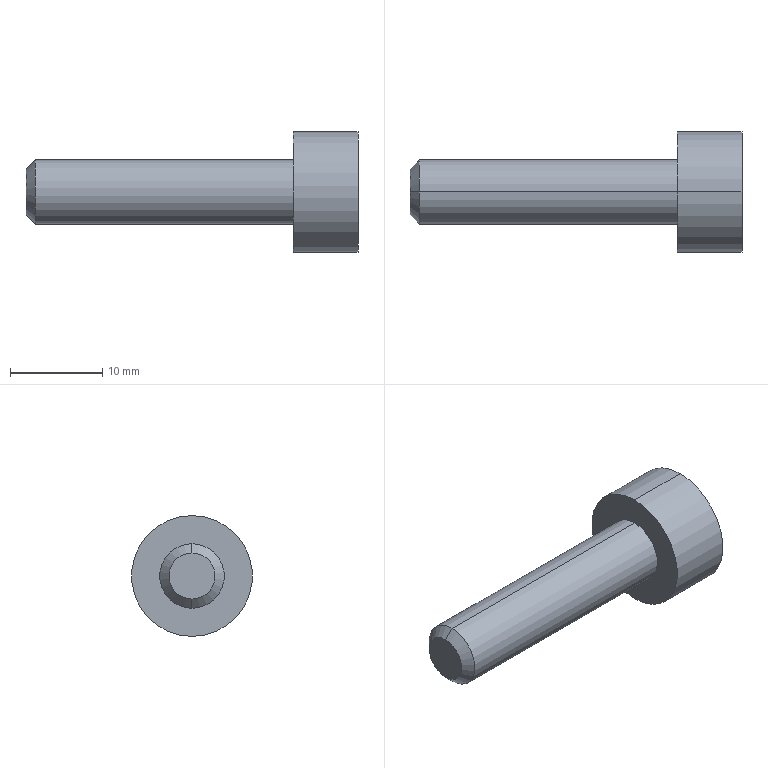Component | SolidWorks | HexSocketScrewM6X15-1 | 1 solid | 16 faces | box 36 x 13.09 x 13.09 mm | volume 1927 mm3 | plane 10 | cylinder 4 | cone 2 | commonest cylinder face diameters 13.093 x2 7 x2
build123d program:
from build123d import *

# Parameters (mm, degrees)
SKETCH2_R           = 3.5
BOSS_EXTRUDE1_DEPTH = 29
SKETCH3_R           = 6.547
BOSS_EXTRUDE2_DEPTH = 7
CHAMFER1_SIZE       = 1
CUT_EXTRUDE1_DEPTH  = 3


with BuildPart() as part:
    # Sketch2 → Boss-Extrude1 (new body)
    with BuildSketch(Plane.XY):
        with Locations((0, 12.224)):
            Circle(SKETCH2_R)
    extrude(amount=-BOSS_EXTRUDE1_DEPTH)

    # Sketch3 → Boss-Extrude2 (add)
    with BuildSketch(Plane.XY):
        with Locations((0, 12.224)):
            Circle(SKETCH3_R)
    extrude(amount=BOSS_EXTRUDE2_DEPTH)

    # Chamfer1
    chamfer1_edges = [part.edges().sort_by_distance(p)[0] for p in [
        (-3.5, 12.224, -29),
    ]]
    chamfer(chamfer1_edges, length=CHAMFER1_SIZE)

    # Sketch4 → Cut-Extrude1 (cut)
    with BuildSketch(Plane.XY.offset(7)):
        Polygon((0.1708, 16.162), (-3.326, 14.341), (-3.496, 10.402), (-0.1708, 8.285), (3.326, 10.106), (3.496, 14.045), align=None)
    extrude(amount=-CUT_EXTRUDE1_DEPTH, mode=Mode.SUBTRACT)


solid = part.part

# Placed as in the assembly
solid = solid.moved(Location((-277, 0, 0), (0, 90, 0)))
STEP:
#1=COLOUR_RGB('',0.7922,0.8196,0.9333);
#2=FILL_AREA_STYLE_COLOUR('',#1);
#3=FILL_AREA_STYLE('',(#2));
#4=SURFACE_STYLE_FILL_AREA(#3);
#5=SURFACE_SIDE_STYLE('',(#4));
#6=SURFACE_STYLE_USAGE(.BOTH.,#5);
#7=PRESENTATION_STYLE_ASSIGNMENT((#6));
#8=CARTESIAN_POINT('',(-12.047,0.4812,0.09843));
#9=VERTEX_POINT('',#8);
#10=CARTESIAN_POINT('',(-12.047,0.4812,-0.09843));
#11=VERTEX_POINT('',#10);
#12=CARTESIAN_POINT('',(-12.047,0.4812,-0.));
#13=DIRECTION('',(-1.,0.,0.));
#14=DIRECTION('',(0.,0.,-1.));
#15=AXIS2_PLACEMENT_3D('',#12,#13,#14);
#16=CIRCLE('',#15,0.09843);
#17=EDGE_CURVE('',#9,#11,#16,.T.);
#18=ORIENTED_EDGE('',*,*,#17,.F.);
#19=CARTESIAN_POINT('',(-12.008,0.4812,0.1378));
#20=VERTEX_POINT('',#19);
#21=CARTESIAN_POINT('',(-12.008,0.4812,0.1378));
#22=DIRECTION('',(0.7071,0.,0.7071));
#23=VECTOR('',#22,39.37);
#24=LINE('',#21,#23);
#25=EDGE_CURVE('',#9,#20,#24,.T.);
#26=ORIENTED_EDGE('',*,*,#25,.T.);
#27=CARTESIAN_POINT('',(-12.008,0.4812,-0.1378));
#28=VERTEX_POINT('',#27);
#29=CARTESIAN_POINT('',(-12.008,0.4812,-0.));
#30=DIRECTION('',(1.,0.,0.));
#31=DIRECTION('',(0.,0.,-1.));
#32=AXIS2_PLACEMENT_3D('',#29,#30,#31);
#33=CIRCLE('',#32,0.1378);
#34=EDGE_CURVE('',#28,#20,#33,.T.);
#35=ORIENTED_EDGE('',*,*,#34,.F.);
#36=CARTESIAN_POINT('',(-12.008,0.4812,-0.1378));
#37=DIRECTION('',(0.7071,0.,-0.7071));
#38=VECTOR('',#37,39.37);
#39=LINE('',#36,#38);
#40=EDGE_CURVE('',#11,#28,#39,.T.);
#41=ORIENTED_EDGE('',*,*,#40,.F.);
#42=EDGE_LOOP('',(#18,#26,#35,#41));
#43=FACE_OUTER_BOUND('',#42,.T.);
#44=CARTESIAN_POINT('',(-12.008,0.4812,-0.));
#45=DIRECTION('',(1.,0.,0.));
#46=DIRECTION('',(0.,0.,-1.));
#47=AXIS2_PLACEMENT_3D('',#44,#45,#46);
#48=CONICAL_SURFACE('',#47,0.1378,0.7854);
#49=ADVANCED_FACE('',(#43),#48,.T.);
#50=CARTESIAN_POINT('',(-10.63,0.4812,-0.2577));
#51=VERTEX_POINT('',#50);
#52=CARTESIAN_POINT('',(-10.63,0.4812,0.2577));
#53=VERTEX_POINT('',#52);
#54=CARTESIAN_POINT('',(-10.63,0.4812,0.));
#55=DIRECTION('',(1.,0.,0.));
#56=DIRECTION('',(0.,0.,-1.));
#57=AXIS2_PLACEMENT_3D('',#54,#55,#56);
#58=CIRCLE('',#57,0.2577);
#59=EDGE_CURVE('',#51,#53,#58,.T.);
#60=ORIENTED_EDGE('',*,*,#59,.F.);
#61=CARTESIAN_POINT('',(-10.906,0.4812,-0.2577));
#62=VERTEX_POINT('',#61);
#63=CARTESIAN_POINT('',(-10.63,0.4812,-0.2577));
#64=DIRECTION('',(-1.,0.,0.));
#65=VECTOR('',#64,39.37);
#66=LINE('',#63,#65);
#67=EDGE_CURVE('',#51,#62,#66,.T.);
#68=ORIENTED_EDGE('',*,*,#67,.T.);
#69=CARTESIAN_POINT('',(-10.906,0.4812,0.2577));
#70=VERTEX_POINT('',#69);
#71=CARTESIAN_POINT('',(-10.906,0.4812,0.));
#72=DIRECTION('',(1.,0.,0.));
#73=DIRECTION('',(0.,0.,-1.));
#74=AXIS2_PLACEMENT_3D('',#71,#72,#73);
#75=CIRCLE('',#74,0.2577);
#76=EDGE_CURVE('',#62,#70,#75,.T.);
#77=ORIENTED_EDGE('',*,*,#76,.T.);
#78=CARTESIAN_POINT('',(-10.63,0.4812,0.2577));
#79=DIRECTION('',(-1.,0.,0.));
#80=VECTOR('',#79,39.37);
#81=LINE('',#78,#80);
#82=EDGE_CURVE('',#53,#70,#81,.T.);
#83=ORIENTED_EDGE('',*,*,#82,.F.);
#84=EDGE_LOOP('',(#60,#68,#77,#83));
#85=FACE_OUTER_BOUND('',#84,.T.);
#86=CARTESIAN_POINT('',(-10.63,0.4812,0.));
#87=DIRECTION('',(-1.,0.,0.));
#88=DIRECTION('',(0.,0.,1.));
#89=AXIS2_PLACEMENT_3D('',#86,#87,#88);
#90=CYLINDRICAL_SURFACE('',#89,0.2577);
#91=ADVANCED_FACE('',(#85),#90,.T.);
#92=ORIENTED_EDGE('',*,*,#34,.T.);
#93=CARTESIAN_POINT('',(-10.906,0.4812,0.1378));
#94=VERTEX_POINT('',#93);
#95=CARTESIAN_POINT('',(-12.047,0.4812,0.1378));
#96=DIRECTION('',(1.,0.,0.));
#97=VECTOR('',#96,39.37);
#98=LINE('',#95,#97);
#99=EDGE_CURVE('',#20,#94,#98,.T.);
#100=ORIENTED_EDGE('',*,*,#99,.T.);
#101=CARTESIAN_POINT('',(-10.906,0.4812,-0.1378));
#102=VERTEX_POINT('',#101);
#103=CARTESIAN_POINT('',(-10.906,0.4812,-0.));
#104=DIRECTION('',(1.,0.,0.));
#105=DIRECTION('',(0.,0.,-1.));
#106=AXIS2_PLACEMENT_3D('',#103,#104,#105);
#107=CIRCLE('',#106,0.1378);
#108=EDGE_CURVE('',#102,#94,#107,.T.);
#109=ORIENTED_EDGE('',*,*,#108,.F.);
#110=CARTESIAN_POINT('',(-12.047,0.4812,-0.1378));
#111=DIRECTION('',(1.,0.,0.));
#112=VECTOR('',#111,39.37);
#113=LINE('',#110,#112);
#114=EDGE_CURVE('',#28,#102,#113,.T.);
#115=ORIENTED_EDGE('',*,*,#114,.F.);
#116=EDGE_LOOP('',(#92,#100,#109,#115));
#117=FACE_OUTER_BOUND('',#116,.T.);
#118=CARTESIAN_POINT('',(-12.047,0.4812,-0.));
#119=DIRECTION('',(1.,0.,0.));
#120=DIRECTION('',(0.,0.,-1.));
#121=AXIS2_PLACEMENT_3D('',#118,#119,#120);
#122=CYLINDRICAL_SURFACE('',#121,0.1378);
#123=ADVANCED_FACE('',(#117),#122,.T.);
#124=ORIENTED_EDGE('',*,*,#99,.F.);
#125=CARTESIAN_POINT('',(-12.008,0.4812,-0.));
#126=DIRECTION('',(1.,0.,0.));
#127=DIRECTION('',(0.,0.,-1.));
#128=AXIS2_PLACEMENT_3D('',#125,#126,#127);
#129=CIRCLE('',#128,0.1378);
#130=EDGE_CURVE('',#20,#28,#129,.T.);
#131=ORIENTED_EDGE('',*,*,#130,.T.);
#132=ORIENTED_EDGE('',*,*,#114,.T.);
#133=CARTESIAN_POINT('',(-10.906,0.4812,-0.));
#134=DIRECTION('',(1.,0.,0.));
#135=DIRECTION('',(0.,0.,-1.));
#136=AXIS2_PLACEMENT_3D('',#133,#134,#135);
#137=CIRCLE('',#136,0.1378);
#138=EDGE_CURVE('',#94,#102,#137,.T.);
#139=ORIENTED_EDGE('',*,*,#138,.F.);
#140=EDGE_LOOP('',(#124,#131,#132,#139));
#141=FACE_OUTER_BOUND('',#140,.T.);
#142=CARTESIAN_POINT('',(-12.047,0.4812,-0.));
#143=DIRECTION('',(1.,0.,0.));
#144=DIRECTION('',(0.,0.,-1.));
#145=AXIS2_PLACEMENT_3D('',#142,#143,#144);
#146=CYLINDRICAL_SURFACE('',#145,0.1378);
#147=ADVANCED_FACE('',(#141),#146,.T.);
#148=CARTESIAN_POINT('',(-12.047,0.4812,-0.));
#149=DIRECTION('',(-1.,0.,0.));
#150=DIRECTION('',(0.,0.,-1.));
#151=AXIS2_PLACEMENT_3D('',#148,#149,#150);
#152=CIRCLE('',#151,0.09843);
#153=EDGE_CURVE('',#11,#9,#152,.T.);
#154=ORIENTED_EDGE('',*,*,#153,.T.);
#155=ORIENTED_EDGE('',*,*,#17,.T.);
#156=EDGE_LOOP('',(#154,#155));
#157=FACE_OUTER_BOUND('',#156,.T.);
#158=CARTESIAN_POINT('',(-12.047,0.4812,-0.));
#159=DIRECTION('',(1.,0.,0.));
#160=DIRECTION('',(0.,0.,-1.));
#161=AXIS2_PLACEMENT_3D('',#158,#159,#160);
#162=PLANE('',#161);
#163=ADVANCED_FACE('',(#157),#162,.F.);
#164=ORIENTED_EDGE('',*,*,#67,.F.);
#165=CARTESIAN_POINT('',(-10.63,0.4812,0.));
#166=DIRECTION('',(1.,0.,0.));
#167=DIRECTION('',(0.,0.,-1.));
#168=AXIS2_PLACEMENT_3D('',#165,#166,#167);
#169=CIRCLE('',#168,0.2577);
#170=EDGE_CURVE('',#53,#51,#169,.T.);
#171=ORIENTED_EDGE('',*,*,#170,.F.);
#172=ORIENTED_EDGE('',*,*,#82,.T.);
#173=CARTESIAN_POINT('',(-10.906,0.4812,0.));
#174=DIRECTION('',(1.,0.,0.));
#175=DIRECTION('',(0.,0.,-1.));
#176=AXIS2_PLACEMENT_3D('',#173,#174,#175);
#177=CIRCLE('',#176,0.2577);
#178=EDGE_CURVE('',#70,#62,#177,.T.);
#179=ORIENTED_EDGE('',*,*,#178,.T.);
#180=EDGE_LOOP('',(#164,#171,#172,#179));
#181=FACE_OUTER_BOUND('',#180,.T.);
#182=CARTESIAN_POINT('',(-10.63,0.4812,0.));
#183=DIRECTION('',(-1.,0.,0.));
#184=DIRECTION('',(0.,0.,1.));
#185=AXIS2_PLACEMENT_3D('',#182,#183,#184);
#186=CYLINDRICAL_SURFACE('',#185,0.2577);
#187=ADVANCED_FACE('',(#181),#186,.T.);
#188=CARTESIAN_POINT('',(-10.63,0.553,-0.1377));
#189=VERTEX_POINT('',#188);
#190=CARTESIAN_POINT('',(-10.63,0.6363,-0.006726));
#191=VERTEX_POINT('',#190);
#192=CARTESIAN_POINT('',(-10.63,0.553,-0.1377));
#193=DIRECTION('',(0.,0.5371,0.8435));
#194=VECTOR('',#193,39.37);
#195=LINE('',#192,#194);
#196=EDGE_CURVE('',#189,#191,#195,.T.);
#197=ORIENTED_EDGE('',*,*,#196,.F.);
#198=CARTESIAN_POINT('',(-10.63,0.3979,-0.1309));
#199=VERTEX_POINT('',#198);
#200=CARTESIAN_POINT('',(-10.63,0.3979,-0.1309));
#201=DIRECTION('',(0.,0.9991,-0.04333));
#202=VECTOR('',#201,39.37);
#203=LINE('',#200,#202);
#204=EDGE_CURVE('',#199,#189,#203,.T.);
#205=ORIENTED_EDGE('',*,*,#204,.F.);
#206=CARTESIAN_POINT('',(-10.63,0.3262,0.006726));
#207=VERTEX_POINT('',#206);
#208=CARTESIAN_POINT('',(-10.63,0.3262,0.006726));
#209=DIRECTION('',(0.,0.462,-0.8869));
#210=VECTOR('',#209,39.37);
#211=LINE('',#208,#210);
#212=EDGE_CURVE('',#207,#199,#211,.T.);
#213=ORIENTED_EDGE('',*,*,#212,.F.);
#214=CARTESIAN_POINT('',(-10.63,0.4095,0.1377));
#215=VERTEX_POINT('',#214);
#216=CARTESIAN_POINT('',(-10.63,0.4095,0.1377));
#217=DIRECTION('',(0.,-0.5371,-0.8435));
#218=VECTOR('',#217,39.37);
#219=LINE('',#216,#218);
#220=EDGE_CURVE('',#215,#207,#219,.T.);
#221=ORIENTED_EDGE('',*,*,#220,.F.);
#222=CARTESIAN_POINT('',(-10.63,0.5646,0.1309));
#223=VERTEX_POINT('',#222);
#224=CARTESIAN_POINT('',(-10.63,0.5646,0.1309));
#225=DIRECTION('',(0.,-0.9991,0.04333));
#226=VECTOR('',#225,39.37);
#227=LINE('',#224,#226);
#228=EDGE_CURVE('',#223,#215,#227,.T.);
#229=ORIENTED_EDGE('',*,*,#228,.F.);
#230=CARTESIAN_POINT('',(-10.63,0.6363,-0.006726));
#231=DIRECTION('',(0.,-0.462,0.8869));
#232=VECTOR('',#231,39.37);
#233=LINE('',#230,#232);
#234=EDGE_CURVE('',#191,#223,#233,.T.);
#235=ORIENTED_EDGE('',*,*,#234,.F.);
#236=EDGE_LOOP('',(#197,#205,#213,#221,#229,#235));
#237=FACE_BOUND('',#236,.T.);
#238=ORIENTED_EDGE('',*,*,#170,.T.);
#239=ORIENTED_EDGE('',*,*,#59,.T.);
#240=EDGE_LOOP('',(#238,#239));
#241=FACE_OUTER_BOUND('',#240,.T.);
#242=CARTESIAN_POINT('',(-10.63,0.4812,0.));
#243=DIRECTION('',(1.,0.,0.));
#244=DIRECTION('',(0.,0.,-1.));
#245=AXIS2_PLACEMENT_3D('',#242,#243,#244);
#246=PLANE('',#245);
#247=ADVANCED_FACE('',(#237,#241),#246,.T.);
#248=ORIENTED_EDGE('',*,*,#108,.T.);
#249=ORIENTED_EDGE('',*,*,#138,.T.);
#250=EDGE_LOOP('',(#248,#249));
#251=FACE_BOUND('',#250,.T.);
#252=ORIENTED_EDGE('',*,*,#178,.F.);
#253=ORIENTED_EDGE('',*,*,#76,.F.);
#254=EDGE_LOOP('',(#252,#253));
#255=FACE_OUTER_BOUND('',#254,.T.);
#256=CARTESIAN_POINT('',(-10.906,0.4812,0.));
#257=DIRECTION('',(1.,0.,0.));
#258=DIRECTION('',(0.,0.,-1.));
#259=AXIS2_PLACEMENT_3D('',#256,#257,#258);
#260=PLANE('',#259);
#261=ADVANCED_FACE('',(#251,#255),#260,.F.);
#262=ORIENTED_EDGE('',*,*,#25,.F.);
#263=ORIENTED_EDGE('',*,*,#153,.F.);
#264=ORIENTED_EDGE('',*,*,#40,.T.);
#265=ORIENTED_EDGE('',*,*,#130,.F.);
#266=EDGE_LOOP('',(#262,#263,#264,#265));
#267=FACE_OUTER_BOUND('',#266,.T.);
#268=CARTESIAN_POINT('',(-12.008,0.4812,-0.));
#269=DIRECTION('',(1.,0.,0.));
#270=DIRECTION('',(0.,0.,-1.));
#271=AXIS2_PLACEMENT_3D('',#268,#269,#270);
#272=CONICAL_SURFACE('',#271,0.1378,0.7854);
#273=ADVANCED_FACE('',(#267),#272,.T.);
#274=ORIENTED_EDGE('',*,*,#196,.T.);
#275=CARTESIAN_POINT('',(-10.748,0.6363,-0.006726));
#276=VERTEX_POINT('',#275);
#277=CARTESIAN_POINT('',(-10.748,0.6363,-0.006726));
#278=DIRECTION('',(1.,0.,0.));
#279=VECTOR('',#278,39.37);
#280=LINE('',#277,#279);
#281=EDGE_CURVE('',#276,#191,#280,.T.);
#282=ORIENTED_EDGE('',*,*,#281,.F.);
#283=CARTESIAN_POINT('',(-10.748,0.553,-0.1377));
#284=VERTEX_POINT('',#283);
#285=CARTESIAN_POINT('',(-10.748,0.553,-0.1377));
#286=DIRECTION('',(0.,0.5371,0.8435));
#287=VECTOR('',#286,39.37);
#288=LINE('',#285,#287);
#289=EDGE_CURVE('',#284,#276,#288,.T.);
#290=ORIENTED_EDGE('',*,*,#289,.F.);
#291=CARTESIAN_POINT('',(-10.748,0.553,-0.1377));
#292=DIRECTION('',(1.,0.,0.));
#293=VECTOR('',#292,39.37);
#294=LINE('',#291,#293);
#295=EDGE_CURVE('',#284,#189,#294,.T.);
#296=ORIENTED_EDGE('',*,*,#295,.T.);
#297=EDGE_LOOP('',(#274,#282,#290,#296));
#298=FACE_OUTER_BOUND('',#297,.T.);
#299=CARTESIAN_POINT('',(-10.748,0.553,-0.1377));
#300=DIRECTION('',(0.,0.8435,-0.5371));
#301=DIRECTION('',(0.,0.5371,0.8435));
#302=AXIS2_PLACEMENT_3D('',#299,#300,#301);
#303=PLANE('',#302);
#304=ADVANCED_FACE('',(#298),#303,.F.);
#305=ORIENTED_EDGE('',*,*,#204,.T.);
#306=ORIENTED_EDGE('',*,*,#295,.F.);
#307=CARTESIAN_POINT('',(-10.748,0.3979,-0.1309));
#308=VERTEX_POINT('',#307);
#309=CARTESIAN_POINT('',(-10.748,0.3979,-0.1309));
#310=DIRECTION('',(0.,0.9991,-0.04333));
#311=VECTOR('',#310,39.37);
#312=LINE('',#309,#311);
#313=EDGE_CURVE('',#308,#284,#312,.T.);
#314=ORIENTED_EDGE('',*,*,#313,.F.);
#315=CARTESIAN_POINT('',(-10.748,0.3979,-0.1309));
#316=DIRECTION('',(1.,0.,0.));
#317=VECTOR('',#316,39.37);
#318=LINE('',#315,#317);
#319=EDGE_CURVE('',#308,#199,#318,.T.);
#320=ORIENTED_EDGE('',*,*,#319,.T.);
#321=EDGE_LOOP('',(#305,#306,#314,#320));
#322=FACE_OUTER_BOUND('',#321,.T.);
#323=CARTESIAN_POINT('',(-10.748,0.3979,-0.1309));
#324=DIRECTION('',(0.,-0.04333,-0.9991));
#325=DIRECTION('',(0.,0.9991,-0.04333));
#326=AXIS2_PLACEMENT_3D('',#323,#324,#325);
#327=PLANE('',#326);
#328=ADVANCED_FACE('',(#322),#327,.F.);
#329=ORIENTED_EDGE('',*,*,#212,.T.);
#330=ORIENTED_EDGE('',*,*,#319,.F.);
#331=CARTESIAN_POINT('',(-10.748,0.3262,0.006726));
#332=VERTEX_POINT('',#331);
#333=CARTESIAN_POINT('',(-10.748,0.3262,0.006726));
#334=DIRECTION('',(0.,0.462,-0.8869));
#335=VECTOR('',#334,39.37);
#336=LINE('',#333,#335);
#337=EDGE_CURVE('',#332,#308,#336,.T.);
#338=ORIENTED_EDGE('',*,*,#337,.F.);
#339=CARTESIAN_POINT('',(-10.748,0.3262,0.006726));
#340=DIRECTION('',(1.,0.,0.));
#341=VECTOR('',#340,39.37);
#342=LINE('',#339,#341);
#343=EDGE_CURVE('',#332,#207,#342,.T.);
#344=ORIENTED_EDGE('',*,*,#343,.T.);
#345=EDGE_LOOP('',(#329,#330,#338,#344));
#346=FACE_OUTER_BOUND('',#345,.T.);
#347=CARTESIAN_POINT('',(-10.748,0.3262,0.006726));
#348=DIRECTION('',(0.,-0.8869,-0.462));
#349=DIRECTION('',(0.,0.462,-0.8869));
#350=AXIS2_PLACEMENT_3D('',#347,#348,#349);
#351=PLANE('',#350);
#352=ADVANCED_FACE('',(#346),#351,.F.);
#353=ORIENTED_EDGE('',*,*,#220,.T.);
#354=ORIENTED_EDGE('',*,*,#343,.F.);
#355=CARTESIAN_POINT('',(-10.748,0.4095,0.1377));
#356=VERTEX_POINT('',#355);
#357=CARTESIAN_POINT('',(-10.748,0.4095,0.1377));
#358=DIRECTION('',(0.,-0.5371,-0.8435));
#359=VECTOR('',#358,39.37);
#360=LINE('',#357,#359);
#361=EDGE_CURVE('',#356,#332,#360,.T.);
#362=ORIENTED_EDGE('',*,*,#361,.F.);
#363=CARTESIAN_POINT('',(-10.748,0.4095,0.1377));
#364=DIRECTION('',(1.,0.,0.));
#365=VECTOR('',#364,39.37);
#366=LINE('',#363,#365);
#367=EDGE_CURVE('',#356,#215,#366,.T.);
#368=ORIENTED_EDGE('',*,*,#367,.T.);
#369=EDGE_LOOP('',(#353,#354,#362,#368));
#370=FACE_OUTER_BOUND('',#369,.T.);
#371=CARTESIAN_POINT('',(-10.748,0.4095,0.1377));
#372=DIRECTION('',(0.,-0.8435,0.5371));
#373=DIRECTION('',(0.,-0.5371,-0.8435));
#374=AXIS2_PLACEMENT_3D('',#371,#372,#373);
#375=PLANE('',#374);
#376=ADVANCED_FACE('',(#370),#375,.F.);
#377=ORIENTED_EDGE('',*,*,#228,.T.);
#378=ORIENTED_EDGE('',*,*,#367,.F.);
#379=CARTESIAN_POINT('',(-10.748,0.5646,0.1309));
#380=VERTEX_POINT('',#379);
#381=CARTESIAN_POINT('',(-10.748,0.5646,0.1309));
#382=DIRECTION('',(0.,-0.9991,0.04333));
#383=VECTOR('',#382,39.37);
#384=LINE('',#381,#383);
#385=EDGE_CURVE('',#380,#356,#384,.T.);
#386=ORIENTED_EDGE('',*,*,#385,.F.);
#387=CARTESIAN_POINT('',(-10.748,0.5646,0.1309));
#388=DIRECTION('',(1.,0.,0.));
#389=VECTOR('',#388,39.37);
#390=LINE('',#387,#389);
#391=EDGE_CURVE('',#380,#223,#390,.T.);
#392=ORIENTED_EDGE('',*,*,#391,.T.);
#393=EDGE_LOOP('',(#377,#378,#386,#392));
#394=FACE_OUTER_BOUND('',#393,.T.);
#395=CARTESIAN_POINT('',(-10.748,0.5646,0.1309));
#396=DIRECTION('',(0.,0.04333,0.9991));
#397=DIRECTION('',(0.,-0.9991,0.04333));
#398=AXIS2_PLACEMENT_3D('',#395,#396,#397);
#399=PLANE('',#398);
#400=ADVANCED_FACE('',(#394),#399,.F.);
#401=ORIENTED_EDGE('',*,*,#234,.T.);
#402=ORIENTED_EDGE('',*,*,#391,.F.);
#403=CARTESIAN_POINT('',(-10.748,0.6363,-0.006726));
#404=DIRECTION('',(0.,-0.462,0.8869));
#405=VECTOR('',#404,39.37);
#406=LINE('',#403,#405);
#407=EDGE_CURVE('',#276,#380,#406,.T.);
#408=ORIENTED_EDGE('',*,*,#407,.F.);
#409=ORIENTED_EDGE('',*,*,#281,.T.);
#410=EDGE_LOOP('',(#401,#402,#408,#409));
#411=FACE_OUTER_BOUND('',#410,.T.);
#412=CARTESIAN_POINT('',(-10.748,0.6363,-0.006726));
#413=DIRECTION('',(0.,0.8869,0.462));
#414=DIRECTION('',(0.,-0.462,0.8869));
#415=AXIS2_PLACEMENT_3D('',#412,#413,#414);
#416=PLANE('',#415);
#417=ADVANCED_FACE('',(#411),#416,.F.);
#418=ORIENTED_EDGE('',*,*,#289,.T.);
#419=ORIENTED_EDGE('',*,*,#407,.T.);
#420=ORIENTED_EDGE('',*,*,#385,.T.);
#421=ORIENTED_EDGE('',*,*,#361,.T.);
#422=ORIENTED_EDGE('',*,*,#337,.T.);
#423=ORIENTED_EDGE('',*,*,#313,.T.);
#424=EDGE_LOOP('',(#418,#419,#420,#421,#422,#423));
#425=FACE_OUTER_BOUND('',#424,.T.);
#426=CARTESIAN_POINT('',(-10.748,0.,0.));
#427=DIRECTION('',(1.,0.,0.));
#428=DIRECTION('',(0.,0.,-1.));
#429=AXIS2_PLACEMENT_3D('',#426,#427,#428);
#430=PLANE('',#429);
#431=ADVANCED_FACE('',(#425),#430,.T.);
#432=CLOSED_SHELL('',(#49,#91,#123,#147,#163,#187,#247,#261,#273,#304,#328,#352,#376,#400,#417,#431));
#433=MANIFOLD_SOLID_BREP('',#432);
#434=STYLED_ITEM('',(#7),#433);
#435=(LENGTH_UNIT()NAMED_UNIT(*)SI_UNIT($,.METRE.));
#436=LENGTH_MEASURE_WITH_UNIT(LENGTH_MEASURE(0.0254),#435);
#437=DIMENSIONAL_EXPONENTS(1.,0.,0.,0.,0.,0.,0.);
#438=(CONVERSION_BASED_UNIT('',#436)LENGTH_UNIT()NAMED_UNIT(#437));
#439=UNCERTAINTY_MEASURE_WITH_UNIT(LENGTH_MEASURE(0.00001),#438,'','');
#440=(NAMED_UNIT(*)PLANE_ANGLE_UNIT()SI_UNIT($,.RADIAN.));
#441=(NAMED_UNIT(*)SI_UNIT($,.STERADIAN.)SOLID_ANGLE_UNIT());
#442=(GEOMETRIC_REPRESENTATION_CONTEXT(3)GLOBAL_UNCERTAINTY_ASSIGNED_CONTEXT((#439))GLOBAL_UNIT_ASSIGNED_CONTEXT((#438,#440,#441))REPRESENTATION_CONTEXT('',''));
#443=MECHANICAL_DESIGN_GEOMETRIC_PRESENTATION_REPRESENTATION('',(#434),#442);
#444=PRESENTATION_LAYER_ASSIGNMENT('','',(#434));
#445=CARTESIAN_POINT('',(0.,0.,0.));
#446=DIRECTION('',(0.,0.,1.));
#447=DIRECTION('',(1.,0.,0.));
#448=AXIS2_PLACEMENT_3D('',#445,#446,#447);
#449=(LENGTH_UNIT()NAMED_UNIT(*)SI_UNIT($,.METRE.));
#450=LENGTH_MEASURE_WITH_UNIT(LENGTH_MEASURE(0.0254),#449);
#451=DIMENSIONAL_EXPONENTS(1.,0.,0.,0.,0.,0.,0.);
#452=(CONVERSION_BASED_UNIT('',#450)LENGTH_UNIT()NAMED_UNIT(#451));
#453=UNCERTAINTY_MEASURE_WITH_UNIT(LENGTH_MEASURE(0.00001),#452,'','');
#454=(NAMED_UNIT(*)PLANE_ANGLE_UNIT()SI_UNIT($,.RADIAN.));
#455=(NAMED_UNIT(*)SI_UNIT($,.STERADIAN.)SOLID_ANGLE_UNIT());
#456=(GEOMETRIC_REPRESENTATION_CONTEXT(3)GLOBAL_UNCERTAINTY_ASSIGNED_CONTEXT((#453))GLOBAL_UNIT_ASSIGNED_CONTEXT((#452,#454,#455))REPRESENTATION_CONTEXT('',''));
#457=ADVANCED_BREP_SHAPE_REPRESENTATION('',(#433,#448),#456);